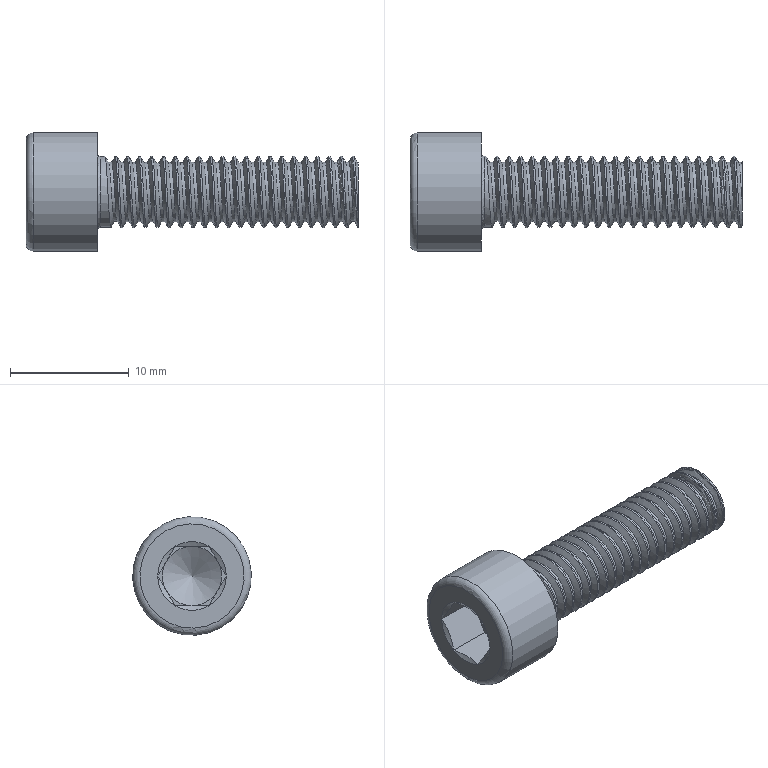Component | NX | M6X20_HEX_BOLT_2 | 1 solid | 30 faces | volume 901 mm3 | plane 16 | cone 7 | cylinder 3 | torus 2 | spline 2 | commonest cylinder face diameters 6 x1 10 x1 5 x1